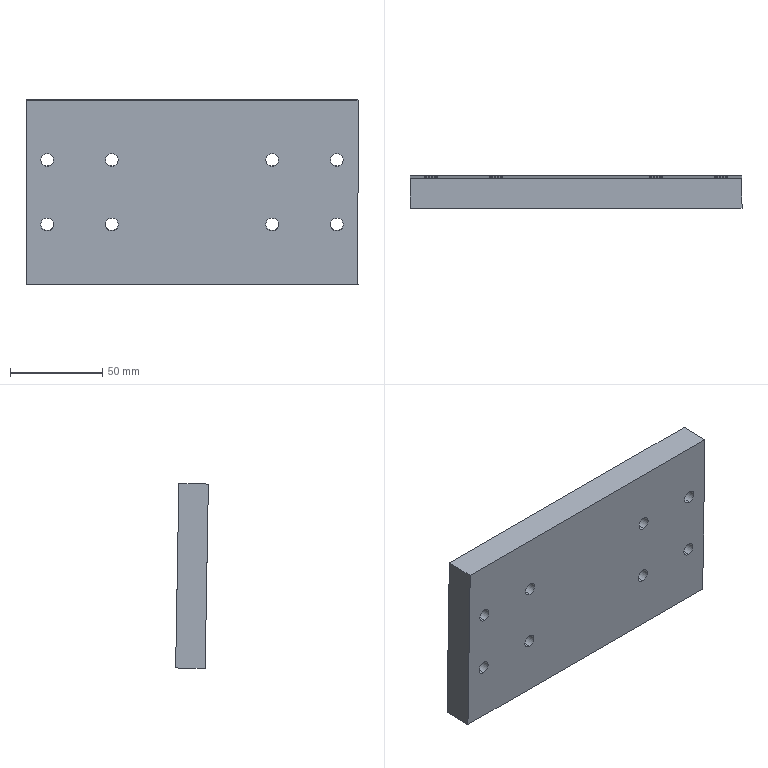Component | SolidWorks | CutterFrontAndRearMovingPlate-3 | 1 solid | 22 faces | box 180 x 17.74 x 100.26 mm | volume 283074 mm3 | cylinder 16 | plane 6 | commonest cylinder face diameters 7 x16
build123d program:
from build123d import *

# Parameters (mm, degrees)
SKETCH1_W           = 100
SKETCH1_H           = 180
BOSS_EXTRUDE1_DEPTH = 16
SKETCH2_R           = 3.5
CUT_EXTRUDE1_DEPTH  = 105.192


with BuildPart() as part:
    # Sketch1 → Boss-Extrude1 (new body)
    with BuildSketch(Plane.XY):
        Rectangle(SKETCH1_W, SKETCH1_H)
    extrude(amount=BOSS_EXTRUDE1_DEPTH)

    # Sketch2 → Cut-Extrude1 (cut, through all)
    with BuildSketch(Plane.XY.offset(16)):
        with Locations((-17.5, 43.5)):
            Circle(SKETCH2_R)
        with Locations((17.5, 43.5)):
            Circle(SKETCH2_R)
        with Locations((17.5, 78.5)):
            Circle(SKETCH2_R)
        with Locations((-17.5, 78.5)):
            Circle(SKETCH2_R)
        with Locations(Location((-17.5, -78.5, 0), (0, 0, 180))):
            Circle(SKETCH2_R)
        with Locations(Location((17.5, -78.5, 0), (0, 0, 180))):
            Circle(SKETCH2_R)
        with Locations(Location((17.5, -43.5, 0), (0, 0, 180))):
            Circle(SKETCH2_R)
        with Locations(Location((-17.5, -43.5, 0), (0, 0, 180))):
            Circle(SKETCH2_R)
    extrude(amount=-CUT_EXTRUDE1_DEPTH, mode=Mode.SUBTRACT)


solid = part.part

# Placed as in the assembly
solid = solid.moved(Location((-17.996, 1224.328, 421.604), (-89, 0, 90)))
STEP:
#1=COLOUR_RGB('',0.7922,0.8196,0.9333);
#2=FILL_AREA_STYLE_COLOUR('',#1);
#3=FILL_AREA_STYLE('',(#2));
#4=SURFACE_STYLE_FILL_AREA(#3);
#5=SURFACE_SIDE_STYLE('',(#4));
#6=SURFACE_STYLE_USAGE(.BOTH.,#5);
#7=PRESENTATION_STYLE_ASSIGNMENT((#6));
#8=CARTESIAN_POINT('',(-2.421,48.817,17.436));
#9=VERTEX_POINT('',#8);
#10=CARTESIAN_POINT('',(-2.421,48.822,17.161));
#11=VERTEX_POINT('',#10);
#12=CARTESIAN_POINT('',(-2.421,48.82,17.298));
#13=DIRECTION('',(0.,-0.9998,-0.01745));
#14=DIRECTION('',(0.,-0.01745,0.9998));
#15=AXIS2_PLACEMENT_3D('',#12,#13,#14);
#16=CIRCLE('',#15,0.1378);
#17=EDGE_CURVE('',#9,#11,#16,.T.);
#18=ORIENTED_EDGE('',*,*,#17,.F.);
#19=CARTESIAN_POINT('',(-2.421,48.187,17.425));
#20=VERTEX_POINT('',#19);
#21=CARTESIAN_POINT('',(-2.421,48.817,17.436));
#22=DIRECTION('',(0.,-0.9998,-0.01745));
#23=VECTOR('',#22,39.37);
#24=LINE('',#21,#23);
#25=EDGE_CURVE('',#9,#20,#24,.T.);
#26=ORIENTED_EDGE('',*,*,#25,.T.);
#27=CARTESIAN_POINT('',(-2.421,48.192,17.15));
#28=VERTEX_POINT('',#27);
#29=CARTESIAN_POINT('',(-2.421,48.19,17.287));
#30=DIRECTION('',(0.,-0.9998,-0.01745));
#31=DIRECTION('',(0.,-0.01745,0.9998));
#32=AXIS2_PLACEMENT_3D('',#29,#30,#31);
#33=CIRCLE('',#32,0.1378);
#34=EDGE_CURVE('',#20,#28,#33,.T.);
#35=ORIENTED_EDGE('',*,*,#34,.T.);
#36=CARTESIAN_POINT('',(-2.421,48.822,17.161));
#37=DIRECTION('',(0.,-0.9998,-0.01745));
#38=VECTOR('',#37,39.37);
#39=LINE('',#36,#38);
#40=EDGE_CURVE('',#11,#28,#39,.T.);
#41=ORIENTED_EDGE('',*,*,#40,.F.);
#42=EDGE_LOOP('',(#18,#26,#35,#41));
#43=FACE_OUTER_BOUND('',#42,.T.);
#44=CARTESIAN_POINT('',(-2.421,48.82,17.298));
#45=DIRECTION('',(0.,-0.9998,-0.01745));
#46=DIRECTION('',(0.,0.01745,-0.9998));
#47=AXIS2_PLACEMENT_3D('',#44,#45,#46);
#48=CYLINDRICAL_SURFACE('',#47,0.1378);
#49=ADVANCED_FACE('',(#43),#48,.F.);
#50=CARTESIAN_POINT('',(-2.421,48.841,16.058));
#51=VERTEX_POINT('',#50);
#52=CARTESIAN_POINT('',(-2.421,48.846,15.783));
#53=VERTEX_POINT('',#52);
#54=CARTESIAN_POINT('',(-2.421,48.844,15.921));
#55=DIRECTION('',(0.,-0.9998,-0.01745));
#56=DIRECTION('',(0.,-0.01745,0.9998));
#57=AXIS2_PLACEMENT_3D('',#54,#55,#56);
#58=CIRCLE('',#57,0.1378);
#59=EDGE_CURVE('',#51,#53,#58,.T.);
#60=ORIENTED_EDGE('',*,*,#59,.F.);
#61=CARTESIAN_POINT('',(-2.421,48.212,16.047));
#62=VERTEX_POINT('',#61);
#63=CARTESIAN_POINT('',(-2.421,48.841,16.058));
#64=DIRECTION('',(0.,-0.9998,-0.01745));
#65=VECTOR('',#64,39.37);
#66=LINE('',#63,#65);
#67=EDGE_CURVE('',#51,#62,#66,.T.);
#68=ORIENTED_EDGE('',*,*,#67,.T.);
#69=CARTESIAN_POINT('',(-2.421,48.216,15.772));
#70=VERTEX_POINT('',#69);
#71=CARTESIAN_POINT('',(-2.421,48.214,15.91));
#72=DIRECTION('',(0.,-0.9998,-0.01745));
#73=DIRECTION('',(0.,-0.01745,0.9998));
#74=AXIS2_PLACEMENT_3D('',#71,#72,#73);
#75=CIRCLE('',#74,0.1378);
#76=EDGE_CURVE('',#62,#70,#75,.T.);
#77=ORIENTED_EDGE('',*,*,#76,.T.);
#78=CARTESIAN_POINT('',(-2.421,48.846,15.783));
#79=DIRECTION('',(0.,-0.9998,-0.01745));
#80=VECTOR('',#79,39.37);
#81=LINE('',#78,#80);
#82=EDGE_CURVE('',#53,#70,#81,.T.);
#83=ORIENTED_EDGE('',*,*,#82,.F.);
#84=EDGE_LOOP('',(#60,#68,#77,#83));
#85=FACE_OUTER_BOUND('',#84,.T.);
#86=CARTESIAN_POINT('',(-2.421,48.844,15.921));
#87=DIRECTION('',(0.,-0.9998,-0.01745));
#88=DIRECTION('',(0.,0.01745,-0.9998));
#89=AXIS2_PLACEMENT_3D('',#86,#87,#88);
#90=CYLINDRICAL_SURFACE('',#89,0.1378);
#91=ADVANCED_FACE('',(#85),#90,.F.);
#92=CARTESIAN_POINT('',(-3.799,48.841,16.058));
#93=VERTEX_POINT('',#92);
#94=CARTESIAN_POINT('',(-3.799,48.846,15.783));
#95=VERTEX_POINT('',#94);
#96=CARTESIAN_POINT('',(-3.799,48.844,15.921));
#97=DIRECTION('',(0.,-0.9998,-0.01745));
#98=DIRECTION('',(0.,-0.01745,0.9998));
#99=AXIS2_PLACEMENT_3D('',#96,#97,#98);
#100=CIRCLE('',#99,0.1378);
#101=EDGE_CURVE('',#93,#95,#100,.T.);
#102=ORIENTED_EDGE('',*,*,#101,.F.);
#103=CARTESIAN_POINT('',(-3.799,48.212,16.047));
#104=VERTEX_POINT('',#103);
#105=CARTESIAN_POINT('',(-3.799,48.841,16.058));
#106=DIRECTION('',(0.,-0.9998,-0.01745));
#107=VECTOR('',#106,39.37);
#108=LINE('',#105,#107);
#109=EDGE_CURVE('',#93,#104,#108,.T.);
#110=ORIENTED_EDGE('',*,*,#109,.T.);
#111=CARTESIAN_POINT('',(-3.799,48.216,15.772));
#112=VERTEX_POINT('',#111);
#113=CARTESIAN_POINT('',(-3.799,48.214,15.91));
#114=DIRECTION('',(0.,-0.9998,-0.01745));
#115=DIRECTION('',(0.,-0.01745,0.9998));
#116=AXIS2_PLACEMENT_3D('',#113,#114,#115);
#117=CIRCLE('',#116,0.1378);
#118=EDGE_CURVE('',#104,#112,#117,.T.);
#119=ORIENTED_EDGE('',*,*,#118,.T.);
#120=CARTESIAN_POINT('',(-3.799,48.846,15.783));
#121=DIRECTION('',(0.,-0.9998,-0.01745));
#122=VECTOR('',#121,39.37);
#123=LINE('',#120,#122);
#124=EDGE_CURVE('',#95,#112,#123,.T.);
#125=ORIENTED_EDGE('',*,*,#124,.F.);
#126=EDGE_LOOP('',(#102,#110,#119,#125));
#127=FACE_OUTER_BOUND('',#126,.T.);
#128=CARTESIAN_POINT('',(-3.799,48.844,15.921));
#129=DIRECTION('',(0.,-0.9998,-0.01745));
#130=DIRECTION('',(0.,0.01745,-0.9998));
#131=AXIS2_PLACEMENT_3D('',#128,#129,#130);
#132=CYLINDRICAL_SURFACE('',#131,0.1378);
#133=ADVANCED_FACE('',(#127),#132,.F.);
#134=CARTESIAN_POINT('',(2.382,48.817,17.436));
#135=VERTEX_POINT('',#134);
#136=CARTESIAN_POINT('',(2.382,48.822,17.161));
#137=VERTEX_POINT('',#136);
#138=CARTESIAN_POINT('',(2.382,48.82,17.298));
#139=DIRECTION('',(0.,-0.9998,-0.01745));
#140=DIRECTION('',(0.,0.01745,-0.9998));
#141=AXIS2_PLACEMENT_3D('',#138,#139,#140);
#142=CIRCLE('',#141,0.1378);
#143=EDGE_CURVE('',#135,#137,#142,.T.);
#144=ORIENTED_EDGE('',*,*,#143,.F.);
#145=CARTESIAN_POINT('',(2.382,48.187,17.425));
#146=VERTEX_POINT('',#145);
#147=CARTESIAN_POINT('',(2.382,48.817,17.436));
#148=DIRECTION('',(0.,-0.9998,-0.01745));
#149=VECTOR('',#148,39.37);
#150=LINE('',#147,#149);
#151=EDGE_CURVE('',#135,#146,#150,.T.);
#152=ORIENTED_EDGE('',*,*,#151,.T.);
#153=CARTESIAN_POINT('',(2.382,48.192,17.15));
#154=VERTEX_POINT('',#153);
#155=CARTESIAN_POINT('',(2.382,48.19,17.287));
#156=DIRECTION('',(0.,-0.9998,-0.01745));
#157=DIRECTION('',(0.,0.01745,-0.9998));
#158=AXIS2_PLACEMENT_3D('',#155,#156,#157);
#159=CIRCLE('',#158,0.1378);
#160=EDGE_CURVE('',#146,#154,#159,.T.);
#161=ORIENTED_EDGE('',*,*,#160,.T.);
#162=CARTESIAN_POINT('',(2.382,48.822,17.161));
#163=DIRECTION('',(0.,-0.9998,-0.01745));
#164=VECTOR('',#163,39.37);
#165=LINE('',#162,#164);
#166=EDGE_CURVE('',#137,#154,#165,.T.);
#167=ORIENTED_EDGE('',*,*,#166,.F.);
#168=EDGE_LOOP('',(#144,#152,#161,#167));
#169=FACE_OUTER_BOUND('',#168,.T.);
#170=CARTESIAN_POINT('',(2.382,48.82,17.298));
#171=DIRECTION('',(0.,-0.9998,-0.01745));
#172=DIRECTION('',(0.,0.01745,-0.9998));
#173=AXIS2_PLACEMENT_3D('',#170,#171,#172);
#174=CYLINDRICAL_SURFACE('',#173,0.1378);
#175=ADVANCED_FACE('',(#169),#174,.F.);
#176=CARTESIAN_POINT('',(2.382,48.841,16.058));
#177=VERTEX_POINT('',#176);
#178=CARTESIAN_POINT('',(2.382,48.846,15.783));
#179=VERTEX_POINT('',#178);
#180=CARTESIAN_POINT('',(2.382,48.844,15.921));
#181=DIRECTION('',(0.,-0.9998,-0.01745));
#182=DIRECTION('',(0.,0.01745,-0.9998));
#183=AXIS2_PLACEMENT_3D('',#180,#181,#182);
#184=CIRCLE('',#183,0.1378);
#185=EDGE_CURVE('',#177,#179,#184,.T.);
#186=ORIENTED_EDGE('',*,*,#185,.F.);
#187=CARTESIAN_POINT('',(2.382,48.212,16.047));
#188=VERTEX_POINT('',#187);
#189=CARTESIAN_POINT('',(2.382,48.841,16.058));
#190=DIRECTION('',(0.,-0.9998,-0.01745));
#191=VECTOR('',#190,39.37);
#192=LINE('',#189,#191);
#193=EDGE_CURVE('',#177,#188,#192,.T.);
#194=ORIENTED_EDGE('',*,*,#193,.T.);
#195=CARTESIAN_POINT('',(2.382,48.216,15.772));
#196=VERTEX_POINT('',#195);
#197=CARTESIAN_POINT('',(2.382,48.214,15.91));
#198=DIRECTION('',(0.,-0.9998,-0.01745));
#199=DIRECTION('',(0.,0.01745,-0.9998));
#200=AXIS2_PLACEMENT_3D('',#197,#198,#199);
#201=CIRCLE('',#200,0.1378);
#202=EDGE_CURVE('',#188,#196,#201,.T.);
#203=ORIENTED_EDGE('',*,*,#202,.T.);
#204=CARTESIAN_POINT('',(2.382,48.846,15.783));
#205=DIRECTION('',(0.,-0.9998,-0.01745));
#206=VECTOR('',#205,39.37);
#207=LINE('',#204,#206);
#208=EDGE_CURVE('',#179,#196,#207,.T.);
#209=ORIENTED_EDGE('',*,*,#208,.F.);
#210=EDGE_LOOP('',(#186,#194,#203,#209));
#211=FACE_OUTER_BOUND('',#210,.T.);
#212=CARTESIAN_POINT('',(2.382,48.844,15.921));
#213=DIRECTION('',(0.,-0.9998,-0.01745));
#214=DIRECTION('',(0.,0.01745,-0.9998));
#215=AXIS2_PLACEMENT_3D('',#212,#213,#214);
#216=CYLINDRICAL_SURFACE('',#215,0.1378);
#217=ADVANCED_FACE('',(#211),#216,.F.);
#218=CARTESIAN_POINT('',(1.004,48.841,16.058));
#219=VERTEX_POINT('',#218);
#220=CARTESIAN_POINT('',(1.004,48.846,15.783));
#221=VERTEX_POINT('',#220);
#222=CARTESIAN_POINT('',(1.004,48.844,15.921));
#223=DIRECTION('',(0.,-0.9998,-0.01745));
#224=DIRECTION('',(0.,0.01745,-0.9998));
#225=AXIS2_PLACEMENT_3D('',#222,#223,#224);
#226=CIRCLE('',#225,0.1378);
#227=EDGE_CURVE('',#219,#221,#226,.T.);
#228=ORIENTED_EDGE('',*,*,#227,.F.);
#229=CARTESIAN_POINT('',(1.004,48.212,16.047));
#230=VERTEX_POINT('',#229);
#231=CARTESIAN_POINT('',(1.004,48.841,16.058));
#232=DIRECTION('',(0.,-0.9998,-0.01745));
#233=VECTOR('',#232,39.37);
#234=LINE('',#231,#233);
#235=EDGE_CURVE('',#219,#230,#234,.T.);
#236=ORIENTED_EDGE('',*,*,#235,.T.);
#237=CARTESIAN_POINT('',(1.004,48.216,15.772));
#238=VERTEX_POINT('',#237);
#239=CARTESIAN_POINT('',(1.004,48.214,15.91));
#240=DIRECTION('',(0.,-0.9998,-0.01745));
#241=DIRECTION('',(0.,0.01745,-0.9998));
#242=AXIS2_PLACEMENT_3D('',#239,#240,#241);
#243=CIRCLE('',#242,0.1378);
#244=EDGE_CURVE('',#230,#238,#243,.T.);
#245=ORIENTED_EDGE('',*,*,#244,.T.);
#246=CARTESIAN_POINT('',(1.004,48.846,15.783));
#247=DIRECTION('',(0.,-0.9998,-0.01745));
#248=VECTOR('',#247,39.37);
#249=LINE('',#246,#248);
#250=EDGE_CURVE('',#221,#238,#249,.T.);
#251=ORIENTED_EDGE('',*,*,#250,.F.);
#252=EDGE_LOOP('',(#228,#236,#245,#251));
#253=FACE_OUTER_BOUND('',#252,.T.);
#254=CARTESIAN_POINT('',(1.004,48.844,15.921));
#255=DIRECTION('',(0.,-0.9998,-0.01745));
#256=DIRECTION('',(0.,0.01745,-0.9998));
#257=AXIS2_PLACEMENT_3D('',#254,#255,#256);
#258=CYLINDRICAL_SURFACE('',#257,0.1378);
#259=ADVANCED_FACE('',(#253),#258,.F.);
#260=CARTESIAN_POINT('',(-3.799,48.817,17.436));
#261=VERTEX_POINT('',#260);
#262=CARTESIAN_POINT('',(-3.799,48.822,17.161));
#263=VERTEX_POINT('',#262);
#264=CARTESIAN_POINT('',(-3.799,48.82,17.298));
#265=DIRECTION('',(0.,-0.9998,-0.01745));
#266=DIRECTION('',(0.,-0.01745,0.9998));
#267=AXIS2_PLACEMENT_3D('',#264,#265,#266);
#268=CIRCLE('',#267,0.1378);
#269=EDGE_CURVE('',#261,#263,#268,.T.);
#270=ORIENTED_EDGE('',*,*,#269,.F.);
#271=CARTESIAN_POINT('',(-3.799,48.187,17.425));
#272=VERTEX_POINT('',#271);
#273=CARTESIAN_POINT('',(-3.799,48.817,17.436));
#274=DIRECTION('',(0.,-0.9998,-0.01745));
#275=VECTOR('',#274,39.37);
#276=LINE('',#273,#275);
#277=EDGE_CURVE('',#261,#272,#276,.T.);
#278=ORIENTED_EDGE('',*,*,#277,.T.);
#279=CARTESIAN_POINT('',(-3.799,48.192,17.15));
#280=VERTEX_POINT('',#279);
#281=CARTESIAN_POINT('',(-3.799,48.19,17.287));
#282=DIRECTION('',(0.,-0.9998,-0.01745));
#283=DIRECTION('',(0.,-0.01745,0.9998));
#284=AXIS2_PLACEMENT_3D('',#281,#282,#283);
#285=CIRCLE('',#284,0.1378);
#286=EDGE_CURVE('',#272,#280,#285,.T.);
#287=ORIENTED_EDGE('',*,*,#286,.T.);
#288=CARTESIAN_POINT('',(-3.799,48.822,17.161));
#289=DIRECTION('',(0.,-0.9998,-0.01745));
#290=VECTOR('',#289,39.37);
#291=LINE('',#288,#290);
#292=EDGE_CURVE('',#263,#280,#291,.T.);
#293=ORIENTED_EDGE('',*,*,#292,.F.);
#294=EDGE_LOOP('',(#270,#278,#287,#293));
#295=FACE_OUTER_BOUND('',#294,.T.);
#296=CARTESIAN_POINT('',(-3.799,48.82,17.298));
#297=DIRECTION('',(0.,-0.9998,-0.01745));
#298=DIRECTION('',(0.,0.01745,-0.9998));
#299=AXIS2_PLACEMENT_3D('',#296,#297,#298);
#300=CYLINDRICAL_SURFACE('',#299,0.1378);
#301=ADVANCED_FACE('',(#295),#300,.F.);
#302=CARTESIAN_POINT('',(1.004,48.817,17.436));
#303=VERTEX_POINT('',#302);
#304=CARTESIAN_POINT('',(1.004,48.822,17.161));
#305=VERTEX_POINT('',#304);
#306=CARTESIAN_POINT('',(1.004,48.82,17.298));
#307=DIRECTION('',(0.,-0.9998,-0.01745));
#308=DIRECTION('',(0.,0.01745,-0.9998));
#309=AXIS2_PLACEMENT_3D('',#306,#307,#308);
#310=CIRCLE('',#309,0.1378);
#311=EDGE_CURVE('',#303,#305,#310,.T.);
#312=ORIENTED_EDGE('',*,*,#311,.F.);
#313=CARTESIAN_POINT('',(1.004,48.187,17.425));
#314=VERTEX_POINT('',#313);
#315=CARTESIAN_POINT('',(1.004,48.817,17.436));
#316=DIRECTION('',(0.,-0.9998,-0.01745));
#317=VECTOR('',#316,39.37);
#318=LINE('',#315,#317);
#319=EDGE_CURVE('',#303,#314,#318,.T.);
#320=ORIENTED_EDGE('',*,*,#319,.T.);
#321=CARTESIAN_POINT('',(1.004,48.192,17.15));
#322=VERTEX_POINT('',#321);
#323=CARTESIAN_POINT('',(1.004,48.19,17.287));
#324=DIRECTION('',(0.,-0.9998,-0.01745));
#325=DIRECTION('',(0.,0.01745,-0.9998));
#326=AXIS2_PLACEMENT_3D('',#323,#324,#325);
#327=CIRCLE('',#326,0.1378);
#328=EDGE_CURVE('',#314,#322,#327,.T.);
#329=ORIENTED_EDGE('',*,*,#328,.T.);
#330=CARTESIAN_POINT('',(1.004,48.822,17.161));
#331=DIRECTION('',(0.,-0.9998,-0.01745));
#332=VECTOR('',#331,39.37);
#333=LINE('',#330,#332);
#334=EDGE_CURVE('',#305,#322,#333,.T.);
#335=ORIENTED_EDGE('',*,*,#334,.F.);
#336=EDGE_LOOP('',(#312,#320,#329,#335));
#337=FACE_OUTER_BOUND('',#336,.T.);
#338=CARTESIAN_POINT('',(1.004,48.82,17.298));
#339=DIRECTION('',(0.,-0.9998,-0.01745));
#340=DIRECTION('',(0.,0.01745,-0.9998));
#341=AXIS2_PLACEMENT_3D('',#338,#339,#340);
#342=CYLINDRICAL_SURFACE('',#341,0.1378);
#343=ADVANCED_FACE('',(#337),#342,.F.);
#344=CARTESIAN_POINT('',(-4.252,48.866,14.641));
#345=VERTEX_POINT('',#344);
#346=CARTESIAN_POINT('',(2.835,48.866,14.641));
#347=VERTEX_POINT('',#346);
#348=CARTESIAN_POINT('',(2.835,48.866,14.641));
#349=DIRECTION('',(1.,0.,-0.));
#350=VECTOR('',#349,39.37);
#351=LINE('',#348,#350);
#352=EDGE_CURVE('',#345,#347,#351,.T.);
#353=ORIENTED_EDGE('',*,*,#352,.T.);
#354=CARTESIAN_POINT('',(2.835,48.236,14.63));
#355=VERTEX_POINT('',#354);
#356=CARTESIAN_POINT('',(2.835,48.236,14.63));
#357=DIRECTION('',(-0.,0.9998,0.01745));
#358=VECTOR('',#357,39.37);
#359=LINE('',#356,#358);
#360=EDGE_CURVE('',#355,#347,#359,.T.);
#361=ORIENTED_EDGE('',*,*,#360,.F.);
#362=CARTESIAN_POINT('',(-4.252,48.236,14.63));
#363=VERTEX_POINT('',#362);
#364=CARTESIAN_POINT('',(2.835,48.236,14.63));
#365=DIRECTION('',(1.,0.,-0.));
#366=VECTOR('',#365,39.37);
#367=LINE('',#364,#366);
#368=EDGE_CURVE('',#363,#355,#367,.T.);
#369=ORIENTED_EDGE('',*,*,#368,.F.);
#370=CARTESIAN_POINT('',(-4.252,48.236,14.63));
#371=DIRECTION('',(-0.,0.9998,0.01745));
#372=VECTOR('',#371,39.37);
#373=LINE('',#370,#372);
#374=EDGE_CURVE('',#363,#345,#373,.T.);
#375=ORIENTED_EDGE('',*,*,#374,.T.);
#376=EDGE_LOOP('',(#353,#361,#369,#375));
#377=FACE_OUTER_BOUND('',#376,.T.);
#378=CARTESIAN_POINT('',(2.835,48.236,14.63));
#379=DIRECTION('',(0.,-0.01745,0.9998));
#380=DIRECTION('',(-1.,-0.,0.));
#381=AXIS2_PLACEMENT_3D('',#378,#379,#380);
#382=PLANE('',#381);
#383=ADVANCED_FACE('',(#377),#382,.F.);
#384=CARTESIAN_POINT('',(2.835,48.797,18.578));
#385=VERTEX_POINT('',#384);
#386=CARTESIAN_POINT('',(2.835,48.797,18.578));
#387=DIRECTION('',(0.,-0.01745,0.9998));
#388=VECTOR('',#387,39.37);
#389=LINE('',#386,#388);
#390=EDGE_CURVE('',#347,#385,#389,.T.);
#391=ORIENTED_EDGE('',*,*,#390,.T.);
#392=CARTESIAN_POINT('',(2.835,48.168,18.567));
#393=VERTEX_POINT('',#392);
#394=CARTESIAN_POINT('',(2.835,48.168,18.567));
#395=DIRECTION('',(-0.,0.9998,0.01745));
#396=VECTOR('',#395,39.37);
#397=LINE('',#394,#396);
#398=EDGE_CURVE('',#393,#385,#397,.T.);
#399=ORIENTED_EDGE('',*,*,#398,.F.);
#400=CARTESIAN_POINT('',(2.835,48.168,18.567));
#401=DIRECTION('',(0.,-0.01745,0.9998));
#402=VECTOR('',#401,39.37);
#403=LINE('',#400,#402);
#404=EDGE_CURVE('',#355,#393,#403,.T.);
#405=ORIENTED_EDGE('',*,*,#404,.F.);
#406=ORIENTED_EDGE('',*,*,#360,.T.);
#407=EDGE_LOOP('',(#391,#399,#405,#406));
#408=FACE_OUTER_BOUND('',#407,.T.);
#409=CARTESIAN_POINT('',(2.835,48.168,18.567));
#410=DIRECTION('',(-1.,-0.,0.));
#411=DIRECTION('',(-0.,0.9998,0.01745));
#412=AXIS2_PLACEMENT_3D('',#409,#410,#411);
#413=PLANE('',#412);
#414=ADVANCED_FACE('',(#408),#413,.F.);
#415=CARTESIAN_POINT('',(-4.252,48.797,18.578));
#416=VERTEX_POINT('',#415);
#417=CARTESIAN_POINT('',(2.835,48.797,18.578));
#418=DIRECTION('',(-1.,-0.,0.));
#419=VECTOR('',#418,39.37);
#420=LINE('',#417,#419);
#421=EDGE_CURVE('',#385,#416,#420,.T.);
#422=ORIENTED_EDGE('',*,*,#421,.T.);
#423=CARTESIAN_POINT('',(-4.252,48.168,18.567));
#424=VERTEX_POINT('',#423);
#425=CARTESIAN_POINT('',(-4.252,48.168,18.567));
#426=DIRECTION('',(-0.,0.9998,0.01745));
#427=VECTOR('',#426,39.37);
#428=LINE('',#425,#427);
#429=EDGE_CURVE('',#424,#416,#428,.T.);
#430=ORIENTED_EDGE('',*,*,#429,.F.);
#431=CARTESIAN_POINT('',(2.835,48.168,18.567));
#432=DIRECTION('',(-1.,-0.,0.));
#433=VECTOR('',#432,39.37);
#434=LINE('',#431,#433);
#435=EDGE_CURVE('',#393,#424,#434,.T.);
#436=ORIENTED_EDGE('',*,*,#435,.F.);
#437=ORIENTED_EDGE('',*,*,#398,.T.);
#438=EDGE_LOOP('',(#422,#430,#436,#437));
#439=FACE_OUTER_BOUND('',#438,.T.);
#440=CARTESIAN_POINT('',(2.835,48.168,18.567));
#441=DIRECTION('',(-0.,0.01745,-0.9998));
#442=DIRECTION('',(1.,0.,-0.));
#443=AXIS2_PLACEMENT_3D('',#440,#441,#442);
#444=PLANE('',#443);
#445=ADVANCED_FACE('',(#439),#444,.F.);
#446=CARTESIAN_POINT('',(-4.252,48.797,18.578));
#447=DIRECTION('',(-0.,0.01745,-0.9998));
#448=VECTOR('',#447,39.37);
#449=LINE('',#446,#448);
#450=EDGE_CURVE('',#416,#345,#449,.T.);
#451=ORIENTED_EDGE('',*,*,#450,.T.);
#452=ORIENTED_EDGE('',*,*,#374,.F.);
#453=CARTESIAN_POINT('',(-4.252,48.168,18.567));
#454=DIRECTION('',(-0.,0.01745,-0.9998));
#455=VECTOR('',#454,39.37);
#456=LINE('',#453,#455);
#457=EDGE_CURVE('',#424,#363,#456,.T.);
#458=ORIENTED_EDGE('',*,*,#457,.F.);
#459=ORIENTED_EDGE('',*,*,#429,.T.);
#460=EDGE_LOOP('',(#451,#452,#458,#459));
#461=FACE_OUTER_BOUND('',#460,.T.);
#462=CARTESIAN_POINT('',(-4.252,48.168,18.567));
#463=DIRECTION('',(1.,0.,-0.));
#464=DIRECTION('',(0.,-0.9998,-0.01745));
#465=AXIS2_PLACEMENT_3D('',#462,#463,#464);
#466=PLANE('',#465);
#467=ADVANCED_FACE('',(#461),#466,.F.);
#468=CARTESIAN_POINT('',(-2.421,48.19,17.287));
#469=DIRECTION('',(0.,-0.9998,-0.01745));
#470=DIRECTION('',(0.,-0.01745,0.9998));
#471=AXIS2_PLACEMENT_3D('',#468,#469,#470);
#472=CIRCLE('',#471,0.1378);
#473=EDGE_CURVE('',#28,#20,#472,.T.);
#474=ORIENTED_EDGE('',*,*,#473,.F.);
#475=ORIENTED_EDGE('',*,*,#34,.F.);
#476=EDGE_LOOP('',(#474,#475));
#477=FACE_BOUND('',#476,.T.);
#478=CARTESIAN_POINT('',(-2.421,48.214,15.91));
#479=DIRECTION('',(0.,-0.9998,-0.01745));
#480=DIRECTION('',(0.,-0.01745,0.9998));
#481=AXIS2_PLACEMENT_3D('',#478,#479,#480);
#482=CIRCLE('',#481,0.1378);
#483=EDGE_CURVE('',#70,#62,#482,.T.);
#484=ORIENTED_EDGE('',*,*,#483,.F.);
#485=ORIENTED_EDGE('',*,*,#76,.F.);
#486=EDGE_LOOP('',(#484,#485));
#487=FACE_BOUND('',#486,.T.);
#488=CARTESIAN_POINT('',(-3.799,48.214,15.91));
#489=DIRECTION('',(0.,-0.9998,-0.01745));
#490=DIRECTION('',(0.,-0.01745,0.9998));
#491=AXIS2_PLACEMENT_3D('',#488,#489,#490);
#492=CIRCLE('',#491,0.1378);
#493=EDGE_CURVE('',#112,#104,#492,.T.);
#494=ORIENTED_EDGE('',*,*,#493,.F.);
#495=ORIENTED_EDGE('',*,*,#118,.F.);
#496=EDGE_LOOP('',(#494,#495));
#497=FACE_BOUND('',#496,.T.);
#498=CARTESIAN_POINT('',(2.382,48.19,17.287));
#499=DIRECTION('',(0.,-0.9998,-0.01745));
#500=DIRECTION('',(0.,0.01745,-0.9998));
#501=AXIS2_PLACEMENT_3D('',#498,#499,#500);
#502=CIRCLE('',#501,0.1378);
#503=EDGE_CURVE('',#154,#146,#502,.T.);
#504=ORIENTED_EDGE('',*,*,#503,.F.);
#505=ORIENTED_EDGE('',*,*,#160,.F.);
#506=EDGE_LOOP('',(#504,#505));
#507=FACE_BOUND('',#506,.T.);
#508=CARTESIAN_POINT('',(2.382,48.214,15.91));
#509=DIRECTION('',(0.,-0.9998,-0.01745));
#510=DIRECTION('',(0.,0.01745,-0.9998));
#511=AXIS2_PLACEMENT_3D('',#508,#509,#510);
#512=CIRCLE('',#511,0.1378);
#513=EDGE_CURVE('',#196,#188,#512,.T.);
#514=ORIENTED_EDGE('',*,*,#513,.F.);
#515=ORIENTED_EDGE('',*,*,#202,.F.);
#516=EDGE_LOOP('',(#514,#515));
#517=FACE_BOUND('',#516,.T.);
#518=CARTESIAN_POINT('',(1.004,48.214,15.91));
#519=DIRECTION('',(0.,-0.9998,-0.01745));
#520=DIRECTION('',(0.,0.01745,-0.9998));
#521=AXIS2_PLACEMENT_3D('',#518,#519,#520);
#522=CIRCLE('',#521,0.1378);
#523=EDGE_CURVE('',#238,#230,#522,.T.);
#524=ORIENTED_EDGE('',*,*,#523,.F.);
#525=ORIENTED_EDGE('',*,*,#244,.F.);
#526=EDGE_LOOP('',(#524,#525));
#527=FACE_BOUND('',#526,.T.);
#528=CARTESIAN_POINT('',(-3.799,48.19,17.287));
#529=DIRECTION('',(0.,-0.9998,-0.01745));
#530=DIRECTION('',(0.,-0.01745,0.9998));
#531=AXIS2_PLACEMENT_3D('',#528,#529,#530);
#532=CIRCLE('',#531,0.1378);
#533=EDGE_CURVE('',#280,#272,#532,.T.);
#534=ORIENTED_EDGE('',*,*,#533,.F.);
#535=ORIENTED_EDGE('',*,*,#286,.F.);
#536=EDGE_LOOP('',(#534,#535));
#537=FACE_BOUND('',#536,.T.);
#538=CARTESIAN_POINT('',(1.004,48.19,17.287));
#539=DIRECTION('',(0.,-0.9998,-0.01745));
#540=DIRECTION('',(0.,0.01745,-0.9998));
#541=AXIS2_PLACEMENT_3D('',#538,#539,#540);
#542=CIRCLE('',#541,0.1378);
#543=EDGE_CURVE('',#322,#314,#542,.T.);
#544=ORIENTED_EDGE('',*,*,#543,.F.);
#545=ORIENTED_EDGE('',*,*,#328,.F.);
#546=EDGE_LOOP('',(#544,#545));
#547=FACE_BOUND('',#546,.T.);
#548=ORIENTED_EDGE('',*,*,#368,.T.);
#549=ORIENTED_EDGE('',*,*,#404,.T.);
#550=ORIENTED_EDGE('',*,*,#435,.T.);
#551=ORIENTED_EDGE('',*,*,#457,.T.);
#552=EDGE_LOOP('',(#548,#549,#550,#551));
#553=FACE_OUTER_BOUND('',#552,.T.);
#554=CARTESIAN_POINT('',(-0.7085,48.202,16.599));
#555=DIRECTION('',(0.,-0.9998,-0.01745));
#556=DIRECTION('',(-0.,0.01745,-0.9998));
#557=AXIS2_PLACEMENT_3D('',#554,#555,#556);
#558=PLANE('',#557);
#559=ADVANCED_FACE('',(#477,#487,#497,#507,#517,#527,#537,#547,#553),#558,.T.);
#560=CARTESIAN_POINT('',(-2.421,48.82,17.298));
#561=DIRECTION('',(0.,-0.9998,-0.01745));
#562=DIRECTION('',(0.,-0.01745,0.9998));
#563=AXIS2_PLACEMENT_3D('',#560,#561,#562);
#564=CIRCLE('',#563,0.1378);
#565=EDGE_CURVE('',#11,#9,#564,.T.);
#566=ORIENTED_EDGE('',*,*,#565,.T.);
#567=ORIENTED_EDGE('',*,*,#17,.T.);
#568=EDGE_LOOP('',(#566,#567));
#569=FACE_BOUND('',#568,.T.);
#570=CARTESIAN_POINT('',(-2.421,48.844,15.921));
#571=DIRECTION('',(0.,-0.9998,-0.01745));
#572=DIRECTION('',(0.,-0.01745,0.9998));
#573=AXIS2_PLACEMENT_3D('',#570,#571,#572);
#574=CIRCLE('',#573,0.1378);
#575=EDGE_CURVE('',#53,#51,#574,.T.);
#576=ORIENTED_EDGE('',*,*,#575,.T.);
#577=ORIENTED_EDGE('',*,*,#59,.T.);
#578=EDGE_LOOP('',(#576,#577));
#579=FACE_BOUND('',#578,.T.);
#580=CARTESIAN_POINT('',(-3.799,48.844,15.921));
#581=DIRECTION('',(0.,-0.9998,-0.01745));
#582=DIRECTION('',(0.,-0.01745,0.9998));
#583=AXIS2_PLACEMENT_3D('',#580,#581,#582);
#584=CIRCLE('',#583,0.1378);
#585=EDGE_CURVE('',#95,#93,#584,.T.);
#586=ORIENTED_EDGE('',*,*,#585,.T.);
#587=ORIENTED_EDGE('',*,*,#101,.T.);
#588=EDGE_LOOP('',(#586,#587));
#589=FACE_BOUND('',#588,.T.);
#590=CARTESIAN_POINT('',(2.382,48.82,17.298));
#591=DIRECTION('',(0.,-0.9998,-0.01745));
#592=DIRECTION('',(0.,0.01745,-0.9998));
#593=AXIS2_PLACEMENT_3D('',#590,#591,#592);
#594=CIRCLE('',#593,0.1378);
#595=EDGE_CURVE('',#137,#135,#594,.T.);
#596=ORIENTED_EDGE('',*,*,#595,.T.);
#597=ORIENTED_EDGE('',*,*,#143,.T.);
#598=EDGE_LOOP('',(#596,#597));
#599=FACE_BOUND('',#598,.T.);
#600=CARTESIAN_POINT('',(2.382,48.844,15.921));
#601=DIRECTION('',(0.,-0.9998,-0.01745));
#602=DIRECTION('',(0.,0.01745,-0.9998));
#603=AXIS2_PLACEMENT_3D('',#600,#601,#602);
#604=CIRCLE('',#603,0.1378);
#605=EDGE_CURVE('',#179,#177,#604,.T.);
#606=ORIENTED_EDGE('',*,*,#605,.T.);
#607=ORIENTED_EDGE('',*,*,#185,.T.);
#608=EDGE_LOOP('',(#606,#607));
#609=FACE_BOUND('',#608,.T.);
#610=CARTESIAN_POINT('',(1.004,48.844,15.921));
#611=DIRECTION('',(0.,-0.9998,-0.01745));
#612=DIRECTION('',(0.,0.01745,-0.9998));
#613=AXIS2_PLACEMENT_3D('',#610,#611,#612);
#614=CIRCLE('',#613,0.1378);
#615=EDGE_CURVE('',#221,#219,#614,.T.);
#616=ORIENTED_EDGE('',*,*,#615,.T.);
#617=ORIENTED_EDGE('',*,*,#227,.T.);
#618=EDGE_LOOP('',(#616,#617));
#619=FACE_BOUND('',#618,.T.);
#620=CARTESIAN_POINT('',(-3.799,48.82,17.298));
#621=DIRECTION('',(0.,-0.9998,-0.01745));
#622=DIRECTION('',(0.,-0.01745,0.9998));
#623=AXIS2_PLACEMENT_3D('',#620,#621,#622);
#624=CIRCLE('',#623,0.1378);
#625=EDGE_CURVE('',#263,#261,#624,.T.);
#626=ORIENTED_EDGE('',*,*,#625,.T.);
#627=ORIENTED_EDGE('',*,*,#269,.T.);
#628=EDGE_LOOP('',(#626,#627));
#629=FACE_BOUND('',#628,.T.);
#630=CARTESIAN_POINT('',(1.004,48.82,17.298));
#631=DIRECTION('',(0.,-0.9998,-0.01745));
#632=DIRECTION('',(0.,0.01745,-0.9998));
#633=AXIS2_PLACEMENT_3D('',#630,#631,#632);
#634=CIRCLE('',#633,0.1378);
#635=EDGE_CURVE('',#305,#303,#634,.T.);
#636=ORIENTED_EDGE('',*,*,#635,.T.);
#637=ORIENTED_EDGE('',*,*,#311,.T.);
#638=EDGE_LOOP('',(#636,#637));
#639=FACE_BOUND('',#638,.T.);
#640=ORIENTED_EDGE('',*,*,#352,.F.);
#641=ORIENTED_EDGE('',*,*,#450,.F.);
#642=ORIENTED_EDGE('',*,*,#421,.F.);
#643=ORIENTED_EDGE('',*,*,#390,.F.);
#644=EDGE_LOOP('',(#640,#641,#642,#643));
#645=FACE_OUTER_BOUND('',#644,.T.);
#646=CARTESIAN_POINT('',(-0.7085,48.832,16.61));
#647=DIRECTION('',(0.,-0.9998,-0.01745));
#648=DIRECTION('',(-0.,0.01745,-0.9998));
#649=AXIS2_PLACEMENT_3D('',#646,#647,#648);
#650=PLANE('',#649);
#651=ADVANCED_FACE('',(#569,#579,#589,#599,#609,#619,#629,#639,#645),#650,.F.);
#652=ORIENTED_EDGE('',*,*,#319,.F.);
#653=ORIENTED_EDGE('',*,*,#635,.F.);
#654=ORIENTED_EDGE('',*,*,#334,.T.);
#655=ORIENTED_EDGE('',*,*,#543,.T.);
#656=EDGE_LOOP('',(#652,#653,#654,#655));
#657=FACE_OUTER_BOUND('',#656,.T.);
#658=CARTESIAN_POINT('',(1.004,48.82,17.298));
#659=DIRECTION('',(0.,-0.9998,-0.01745));
#660=DIRECTION('',(0.,0.01745,-0.9998));
#661=AXIS2_PLACEMENT_3D('',#658,#659,#660);
#662=CYLINDRICAL_SURFACE('',#661,0.1378);
#663=ADVANCED_FACE('',(#657),#662,.F.);
#664=ORIENTED_EDGE('',*,*,#277,.F.);
#665=ORIENTED_EDGE('',*,*,#625,.F.);
#666=ORIENTED_EDGE('',*,*,#292,.T.);
#667=ORIENTED_EDGE('',*,*,#533,.T.);
#668=EDGE_LOOP('',(#664,#665,#666,#667));
#669=FACE_OUTER_BOUND('',#668,.T.);
#670=CARTESIAN_POINT('',(-3.799,48.82,17.298));
#671=DIRECTION('',(0.,-0.9998,-0.01745));
#672=DIRECTION('',(0.,0.01745,-0.9998));
#673=AXIS2_PLACEMENT_3D('',#670,#671,#672);
#674=CYLINDRICAL_SURFACE('',#673,0.1378);
#675=ADVANCED_FACE('',(#669),#674,.F.);
#676=ORIENTED_EDGE('',*,*,#235,.F.);
#677=ORIENTED_EDGE('',*,*,#615,.F.);
#678=ORIENTED_EDGE('',*,*,#250,.T.);
#679=ORIENTED_EDGE('',*,*,#523,.T.);
#680=EDGE_LOOP('',(#676,#677,#678,#679));
#681=FACE_OUTER_BOUND('',#680,.T.);
#682=CARTESIAN_POINT('',(1.004,48.844,15.921));
#683=DIRECTION('',(0.,-0.9998,-0.01745));
#684=DIRECTION('',(0.,0.01745,-0.9998));
#685=AXIS2_PLACEMENT_3D('',#682,#683,#684);
#686=CYLINDRICAL_SURFACE('',#685,0.1378);
#687=ADVANCED_FACE('',(#681),#686,.F.);
#688=ORIENTED_EDGE('',*,*,#193,.F.);
#689=ORIENTED_EDGE('',*,*,#605,.F.);
#690=ORIENTED_EDGE('',*,*,#208,.T.);
#691=ORIENTED_EDGE('',*,*,#513,.T.);
#692=EDGE_LOOP('',(#688,#689,#690,#691));
#693=FACE_OUTER_BOUND('',#692,.T.);
#694=CARTESIAN_POINT('',(2.382,48.844,15.921));
#695=DIRECTION('',(0.,-0.9998,-0.01745));
#696=DIRECTION('',(0.,0.01745,-0.9998));
#697=AXIS2_PLACEMENT_3D('',#694,#695,#696);
#698=CYLINDRICAL_SURFACE('',#697,0.1378);
#699=ADVANCED_FACE('',(#693),#698,.F.);
#700=ORIENTED_EDGE('',*,*,#151,.F.);
#701=ORIENTED_EDGE('',*,*,#595,.F.);
#702=ORIENTED_EDGE('',*,*,#166,.T.);
#703=ORIENTED_EDGE('',*,*,#503,.T.);
#704=EDGE_LOOP('',(#700,#701,#702,#703));
#705=FACE_OUTER_BOUND('',#704,.T.);
#706=CARTESIAN_POINT('',(2.382,48.82,17.298));
#707=DIRECTION('',(0.,-0.9998,-0.01745));
#708=DIRECTION('',(0.,0.01745,-0.9998));
#709=AXIS2_PLACEMENT_3D('',#706,#707,#708);
#710=CYLINDRICAL_SURFACE('',#709,0.1378);
#711=ADVANCED_FACE('',(#705),#710,.F.);
#712=ORIENTED_EDGE('',*,*,#109,.F.);
#713=ORIENTED_EDGE('',*,*,#585,.F.);
#714=ORIENTED_EDGE('',*,*,#124,.T.);
#715=ORIENTED_EDGE('',*,*,#493,.T.);
#716=EDGE_LOOP('',(#712,#713,#714,#715));
#717=FACE_OUTER_BOUND('',#716,.T.);
#718=CARTESIAN_POINT('',(-3.799,48.844,15.921));
#719=DIRECTION('',(0.,-0.9998,-0.01745));
#720=DIRECTION('',(0.,0.01745,-0.9998));
#721=AXIS2_PLACEMENT_3D('',#718,#719,#720);
#722=CYLINDRICAL_SURFACE('',#721,0.1378);
#723=ADVANCED_FACE('',(#717),#722,.F.);
#724=ORIENTED_EDGE('',*,*,#67,.F.);
#725=ORIENTED_EDGE('',*,*,#575,.F.);
#726=ORIENTED_EDGE('',*,*,#82,.T.);
#727=ORIENTED_EDGE('',*,*,#483,.T.);
#728=EDGE_LOOP('',(#724,#725,#726,#727));
#729=FACE_OUTER_BOUND('',#728,.T.);
#730=CARTESIAN_POINT('',(-2.421,48.844,15.921));
#731=DIRECTION('',(0.,-0.9998,-0.01745));
#732=DIRECTION('',(0.,0.01745,-0.9998));
#733=AXIS2_PLACEMENT_3D('',#730,#731,#732);
#734=CYLINDRICAL_SURFACE('',#733,0.1378);
#735=ADVANCED_FACE('',(#729),#734,.F.);
#736=ORIENTED_EDGE('',*,*,#25,.F.);
#737=ORIENTED_EDGE('',*,*,#565,.F.);
#738=ORIENTED_EDGE('',*,*,#40,.T.);
#739=ORIENTED_EDGE('',*,*,#473,.T.);
#740=EDGE_LOOP('',(#736,#737,#738,#739));
#741=FACE_OUTER_BOUND('',#740,.T.);
#742=CARTESIAN_POINT('',(-2.421,48.82,17.298));
#743=DIRECTION('',(0.,-0.9998,-0.01745));
#744=DIRECTION('',(0.,0.01745,-0.9998));
#745=AXIS2_PLACEMENT_3D('',#742,#743,#744);
#746=CYLINDRICAL_SURFACE('',#745,0.1378);
#747=ADVANCED_FACE('',(#741),#746,.F.);
#748=CLOSED_SHELL('',(#49,#91,#133,#175,#217,#259,#301,#343,#383,#414,#445,#467,#559,#651,#663,#675,#687,#699,#711,#723,#735,#747));
#749=MANIFOLD_SOLID_BREP('',#748);
#750=STYLED_ITEM('',(#7),#749);
#751=PRESENTATION_LAYER_ASSIGNMENT('','',(#750));
#752=(LENGTH_UNIT()NAMED_UNIT(*)SI_UNIT($,.METRE.));
#753=LENGTH_MEASURE_WITH_UNIT(LENGTH_MEASURE(0.0254),#752);
#754=DIMENSIONAL_EXPONENTS(1.,0.,0.,0.,0.,0.,0.);
#755=(CONVERSION_BASED_UNIT('',#753)LENGTH_UNIT()NAMED_UNIT(#754));
#756=UNCERTAINTY_MEASURE_WITH_UNIT(LENGTH_MEASURE(0.00001),#755,'','');
#757=(NAMED_UNIT(*)PLANE_ANGLE_UNIT()SI_UNIT($,.RADIAN.));
#758=(NAMED_UNIT(*)SI_UNIT($,.STERADIAN.)SOLID_ANGLE_UNIT());
#759=(GEOMETRIC_REPRESENTATION_CONTEXT(3)GLOBAL_UNCERTAINTY_ASSIGNED_CONTEXT((#756))GLOBAL_UNIT_ASSIGNED_CONTEXT((#755,#757,#758))REPRESENTATION_CONTEXT('',''));
#760=MECHANICAL_DESIGN_GEOMETRIC_PRESENTATION_REPRESENTATION('',(#750),#759);
#761=CARTESIAN_POINT('',(0.,0.,0.));
#762=DIRECTION('',(0.,0.,1.));
#763=DIRECTION('',(1.,0.,0.));
#764=AXIS2_PLACEMENT_3D('',#761,#762,#763);
#765=(LENGTH_UNIT()NAMED_UNIT(*)SI_UNIT($,.METRE.));
#766=LENGTH_MEASURE_WITH_UNIT(LENGTH_MEASURE(0.0254),#765);
#767=DIMENSIONAL_EXPONENTS(1.,0.,0.,0.,0.,0.,0.);
#768=(CONVERSION_BASED_UNIT('',#766)LENGTH_UNIT()NAMED_UNIT(#767));
#769=UNCERTAINTY_MEASURE_WITH_UNIT(LENGTH_MEASURE(0.00001),#768,'','');
#770=(NAMED_UNIT(*)PLANE_ANGLE_UNIT()SI_UNIT($,.RADIAN.));
#771=(NAMED_UNIT(*)SI_UNIT($,.STERADIAN.)SOLID_ANGLE_UNIT());
#772=(GEOMETRIC_REPRESENTATION_CONTEXT(3)GLOBAL_UNCERTAINTY_ASSIGNED_CONTEXT((#769))GLOBAL_UNIT_ASSIGNED_CONTEXT((#768,#770,#771))REPRESENTATION_CONTEXT('',''));
#773=ADVANCED_BREP_SHAPE_REPRESENTATION('',(#749,#764),#772);